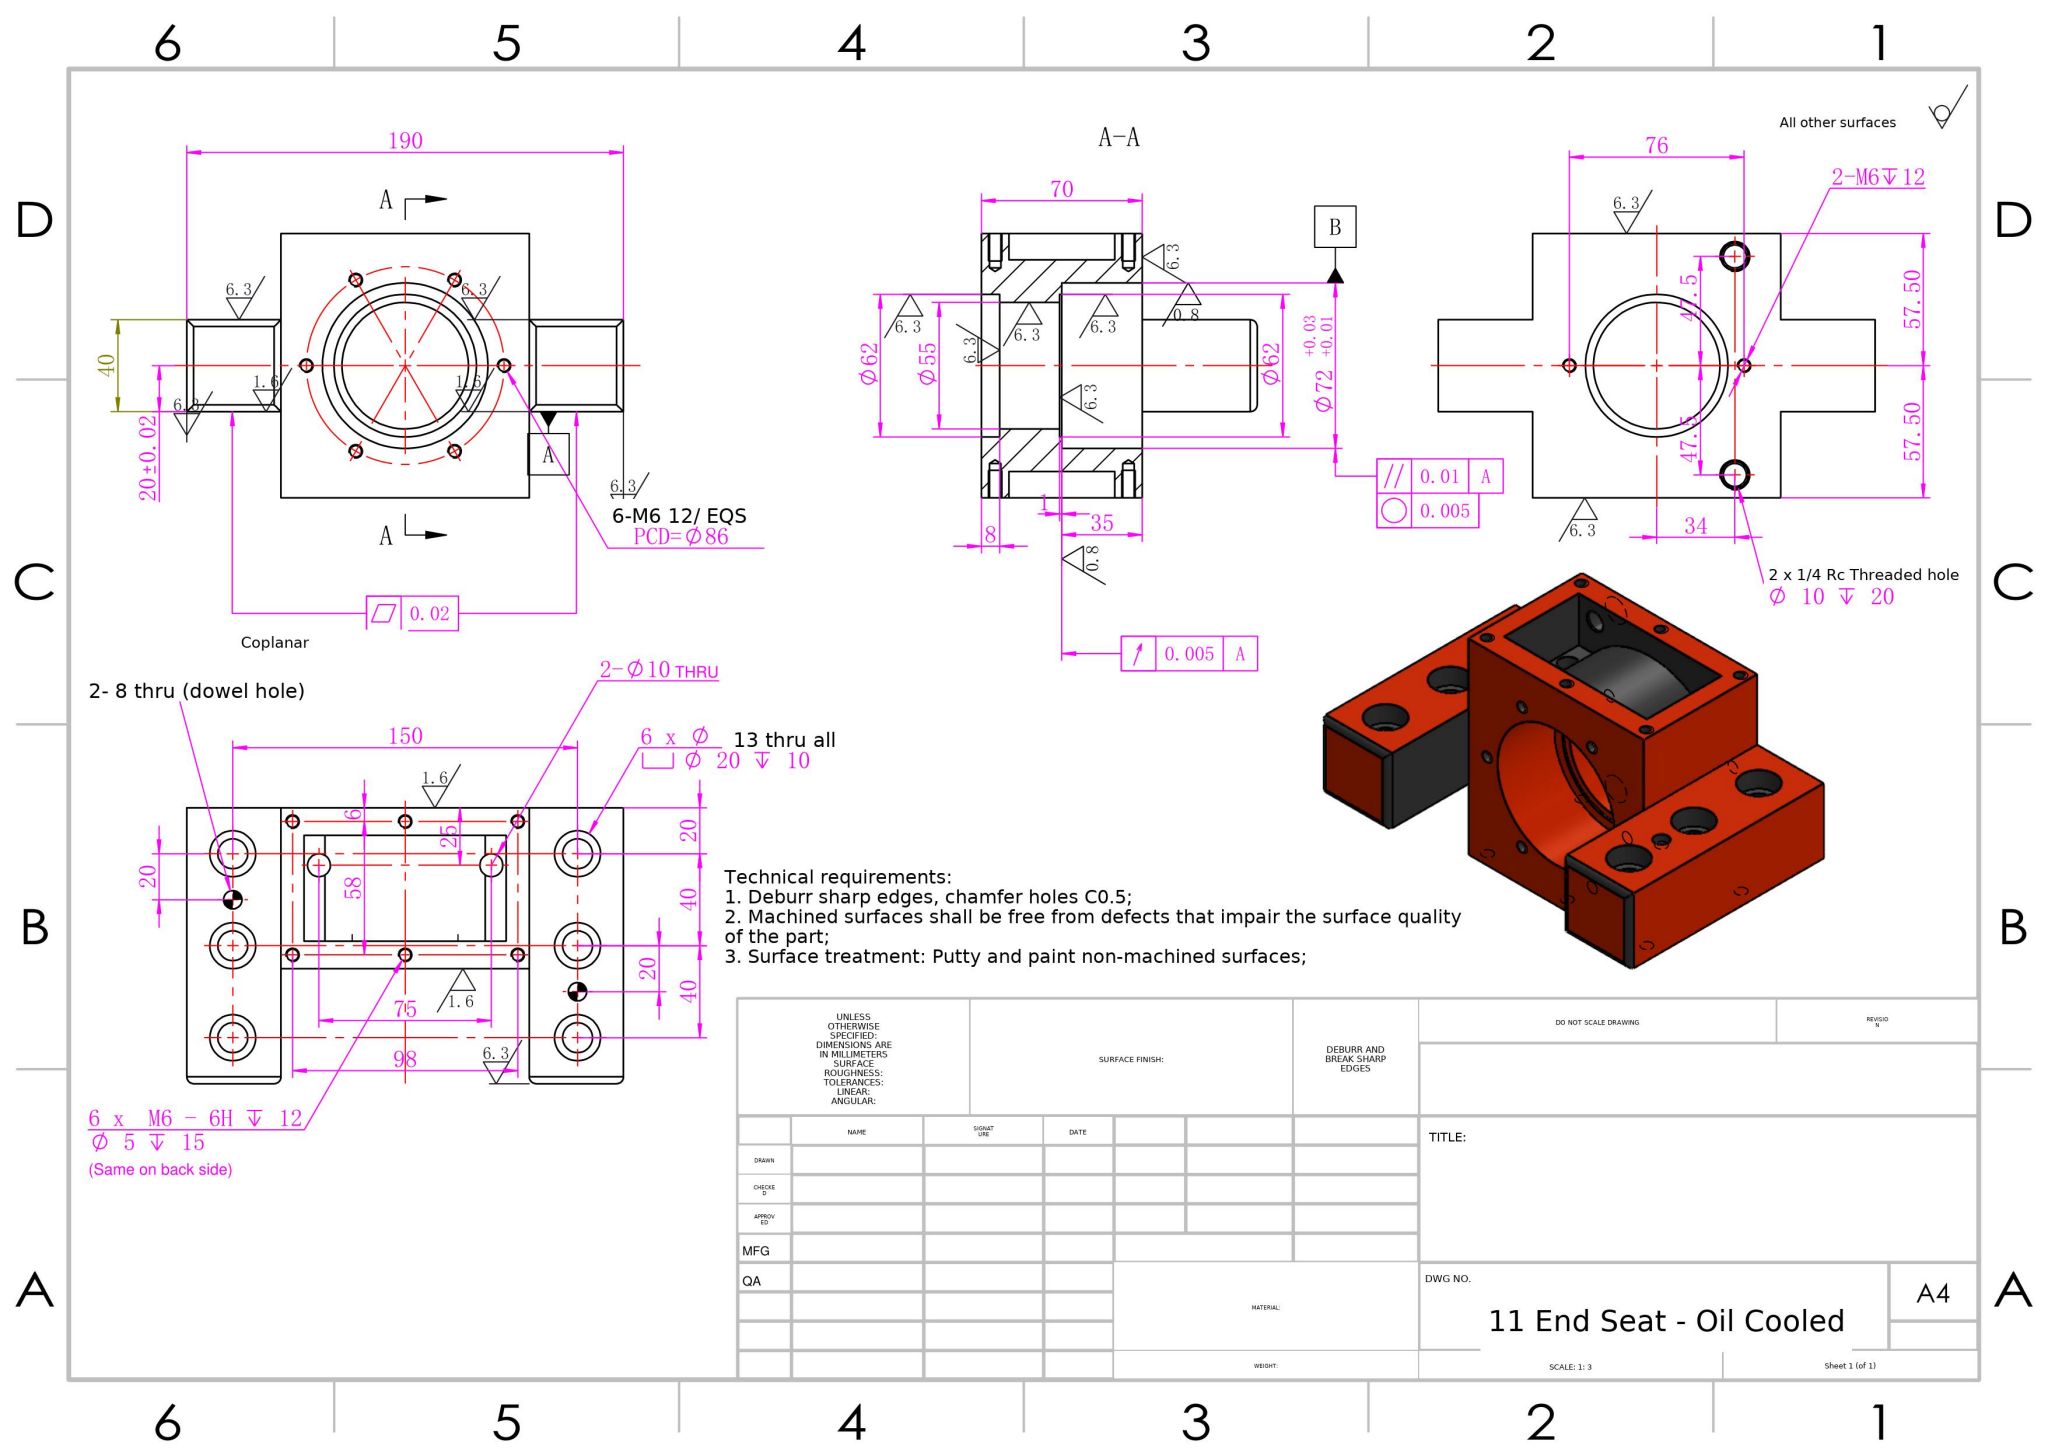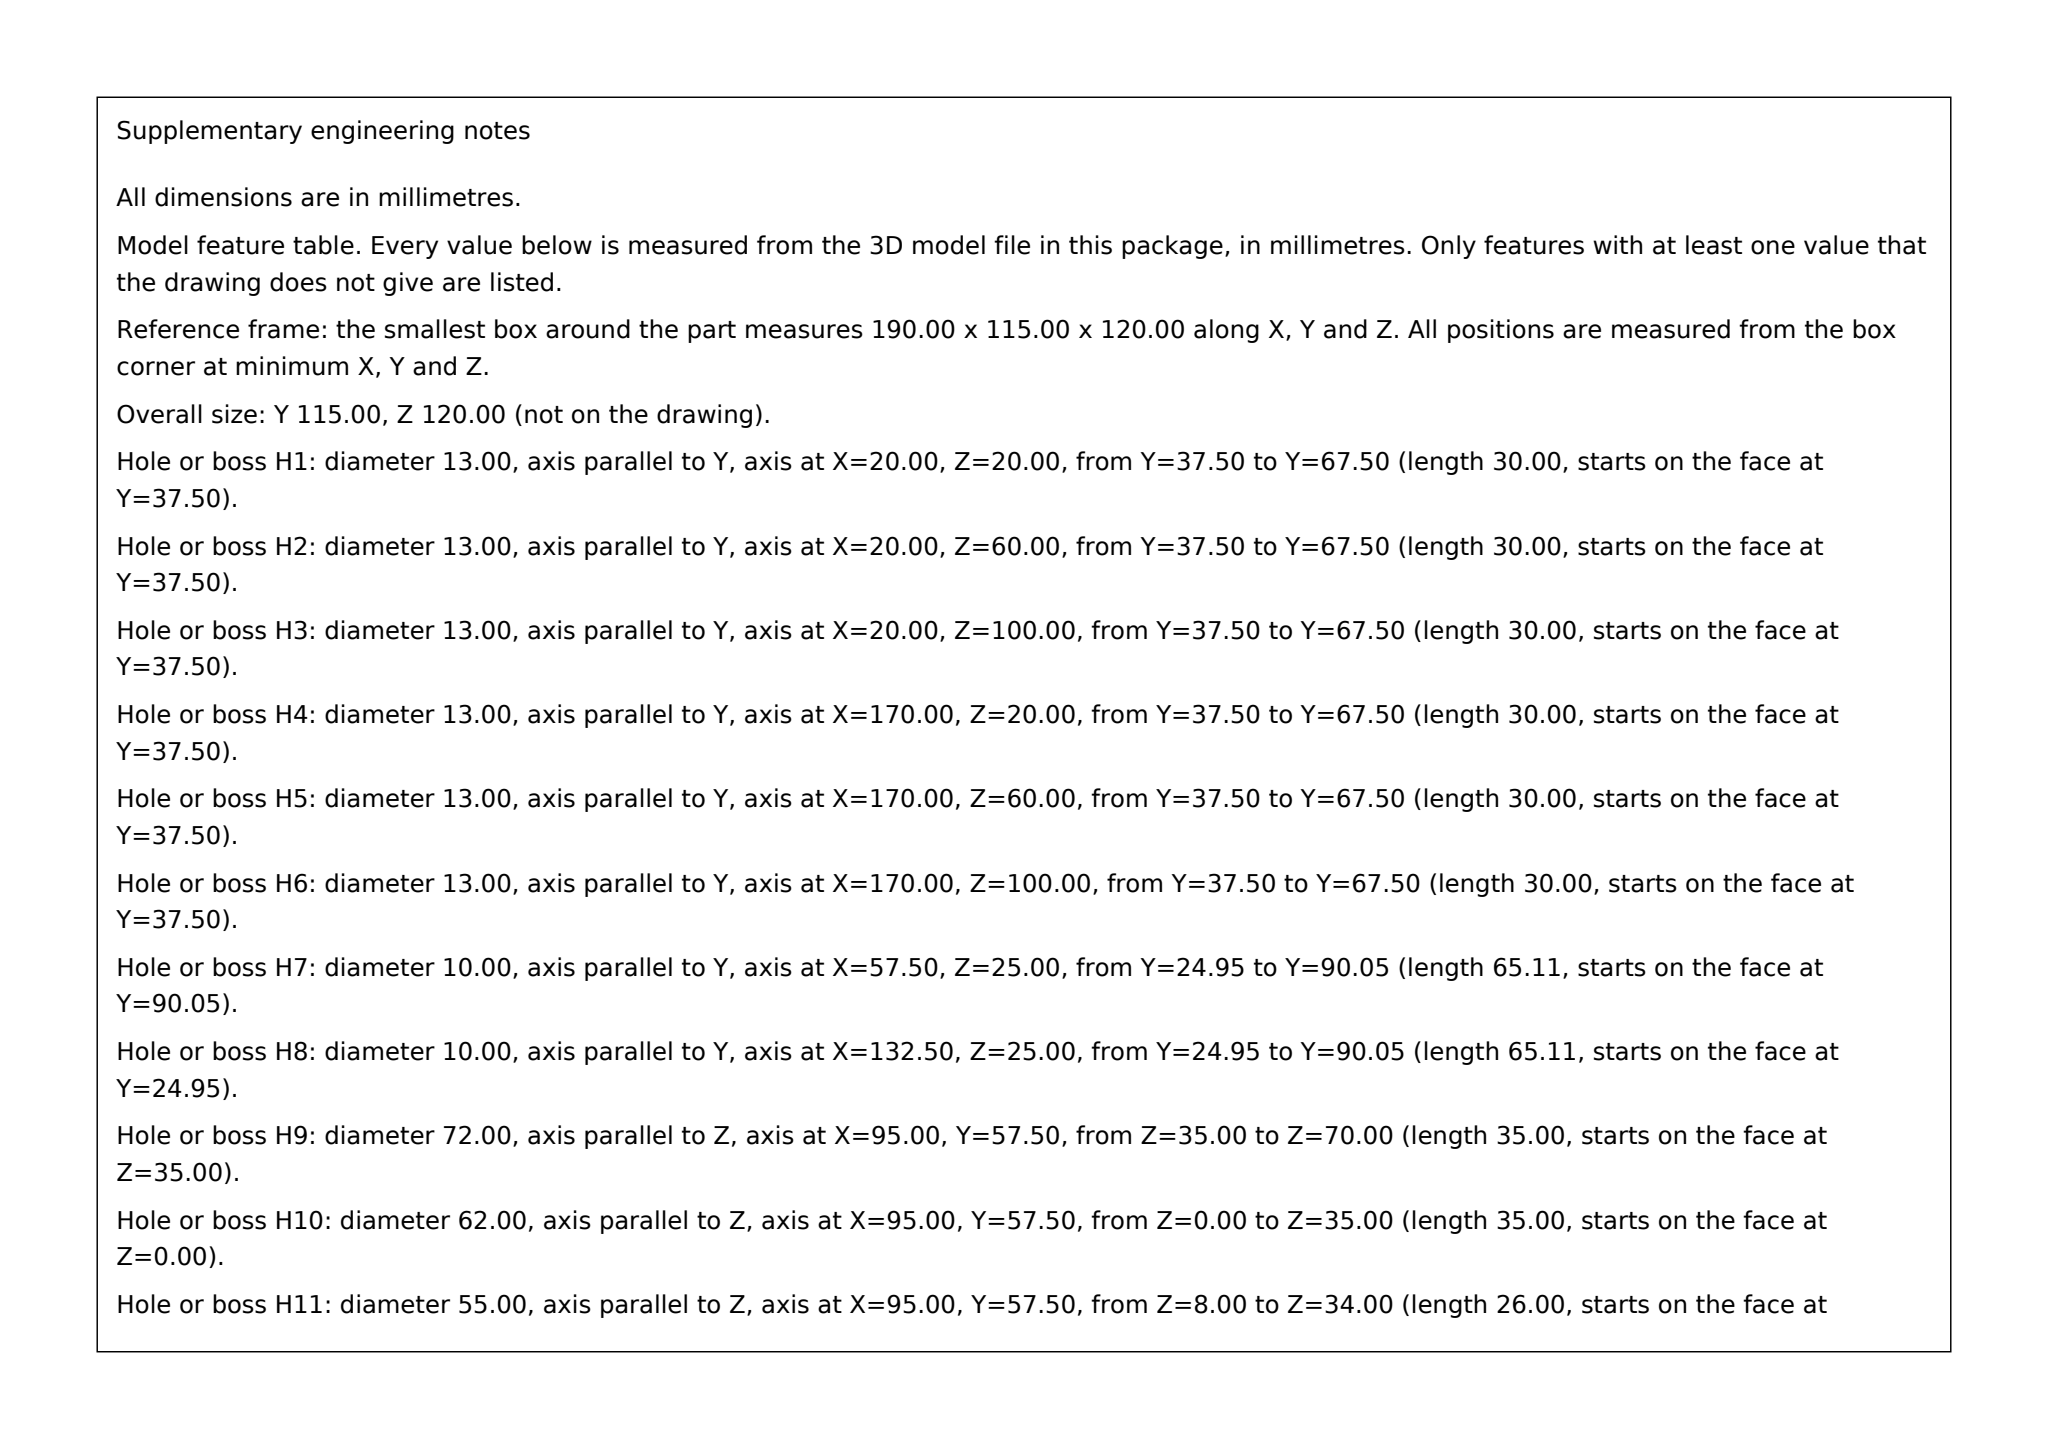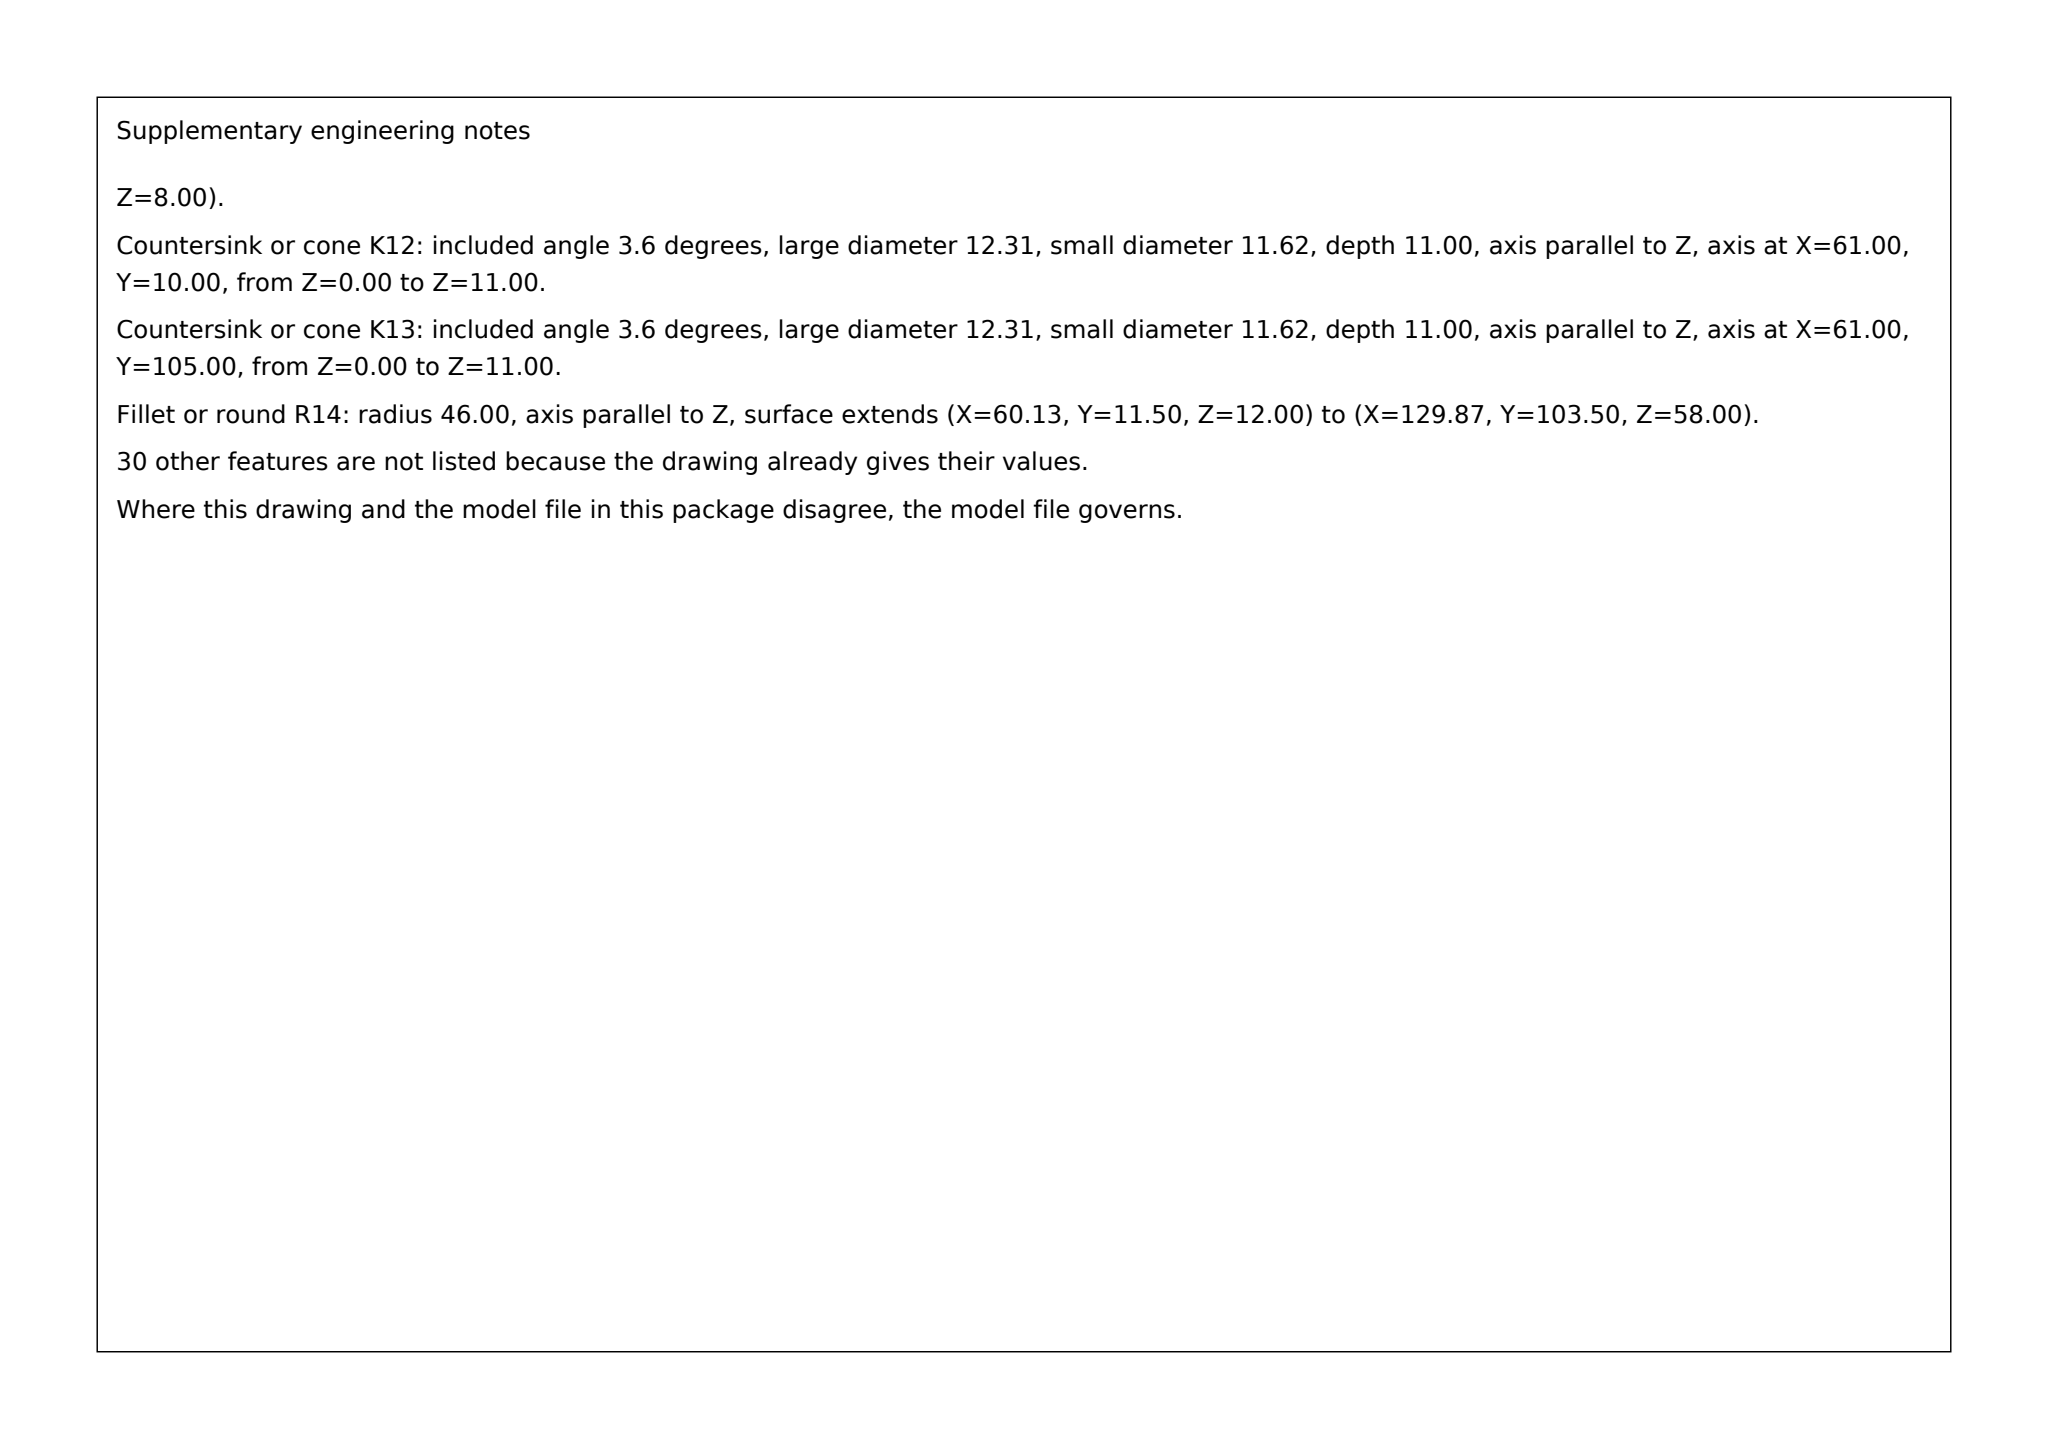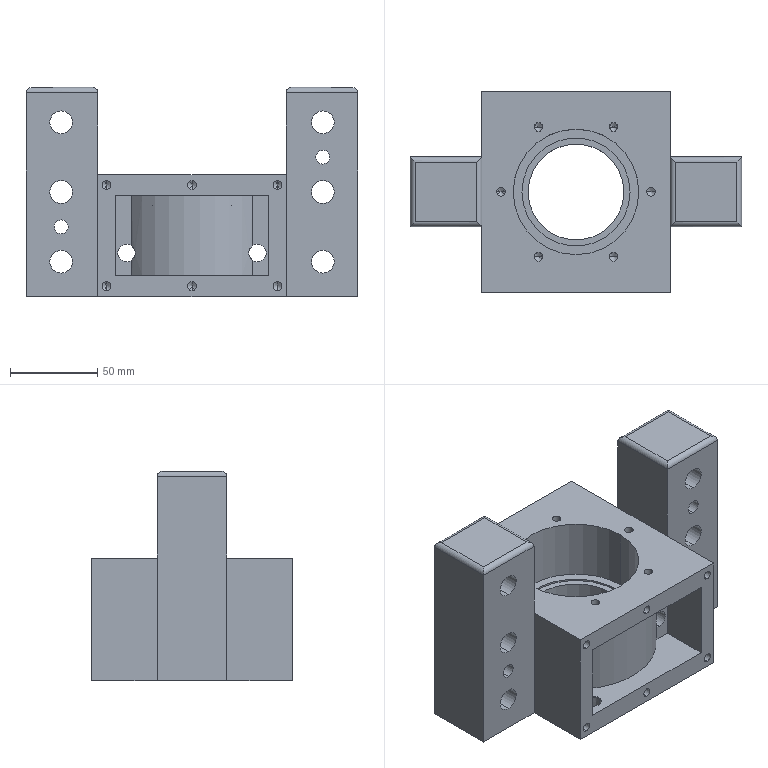Part | SolidWorks | mm | 1 solid | 179 faces | box 190 x 115 x 120 mm | volume 814112 mm3 | cylinder 94 | cone 44 | plane 41 | commonest cylinder face diameters 5 x40 20 x12 13 x12 10 x8 6 x8 8 x4 62 x4 72 x2
build123d program:
from build123d import *

# Parameters (mm, degrees)
SKETCH1_R                                            = 27.5
BOSS_EXTRUDE1_DEPTH                                  = 120
SKETCH3_W                                            = 108
SKETCH3_H                                            = 150
CUT_EXTRUDE1_DEPTH                                   = 50
SKETCH4_R                                            = 36
CUT_EXTRUDE2_DEPTH                                   = 35
SKETCH18_R                                           = 31
CUT_EXTRUDE7_DEPTH                                   = 8
CUT_EXTRUDE8_START                                   = -1
SKETCH19_R                                           = 31
CUT_EXTRUDE8_DEPTH                                   = 1
CYLINDRICAL_COUNTERSUNK_HOLE_FOR_M12_HEX_D           = 13
CYLINDRICAL_COUNTERSUNK_HOLE_FOR_M12_HEX_CBORE_D     = 20
CYLINDRICAL_COUNTERSUNK_HOLE_FOR_M12_HEX_CBORE_DEPTH = 10
CIRPATTERN1_COUNT                                    = 6
SIZE_MM_DOWEL_PIN_HOLE1_D                            = 8
M6_TAPPED_HOLE2_D                                    = 5
M6_TAPPED_HOLE2_DEPTH                                = 18
M6_TAPPED_HOLE2_TIP                                  = 1.502
BOSS_EXTRUDE2_REACH                                  = 187.607
SKETCH23_W                                           = 108
SKETCH23_H                                           = 70
BOSS_EXTRUDE3_REACH                                  = 193.442
SKETCH24_W                                           = 108
SKETCH24_H                                           = 70
SKETCH25_W                                           = 88
SKETCH25_H                                           = 46
CUT_EXTRUDE9_DEPTH                                   = 10
CUT_EXTRUDE10_DEPTH                                  = 46
SKETCH27_R                                           = 5
CUT_EXTRUDE11_DEPTH                                  = 192.442
M6_TAPPED_HOLE3_D                                    = 5
M6_TAPPED_HOLE3_DEPTH                                = 15
M6_TAPPED_HOLE3_TIP                                  = 1.502
M6_TAPPED_HOLE4_D                                    = 5
M6_TAPPED_HOLE4_DEPTH                                = 15
M6_TAPPED_HOLE4_TIP                                  = 1.502
F_1_4_RC_TAPPED_HOLE1_AT_2_COUNT                     = 2
F_1_4_RC_TAPPED_HOLE1_AT_2_PITCH                     = 95
FILLET1_R                                            = 3


with BuildPart() as part:
    # Sketch1 → Boss-Extrude1 (new body)
    with BuildSketch(Plane.XY):
        with BuildLine():
            Line((-95, 20), (-51.235, 20))
            ThreePointArc((-51.235, 20), (-41.806, 35.738), (-27.726, 47.5))
            Line((-27.726, 47.5), (27.726, 47.5))
            ThreePointArc((27.726, 47.5), (41.806, 35.738), (51.235, 20))
            Line((51.235, 20), (95, 20))
            Line((95, 20), (95, -20))
            Line((95, -20), (51.235, -20))
            ThreePointArc((51.235, -20), (41.806, -35.738), (27.726, -47.5))
            Line((27.726, -47.5), (-27.726, -47.5))
            ThreePointArc((-27.726, -47.5), (-41.806, -35.738), (-51.235, -20))
            Line((-51.235, -20), (-95, -20))
            Line((-95, -20), (-95, 20))
        make_face()
        Circle(SKETCH1_R, mode=Mode.SUBTRACT)
    extrude(amount=BOSS_EXTRUDE1_DEPTH)

    # Sketch3 → Cut-Extrude1 (cut)
    with BuildSketch(Plane.XY.offset(120)):
        Rectangle(SKETCH3_W, SKETCH3_H)
    extrude(amount=-CUT_EXTRUDE1_DEPTH, mode=Mode.SUBTRACT)

    # Sketch4 → Cut-Extrude2 (cut)
    with BuildSketch(Plane.XY.offset(70)):
        Circle(SKETCH4_R)
    extrude(amount=-CUT_EXTRUDE2_DEPTH, mode=Mode.SUBTRACT)

    # Sketch18 → Cut-Extrude7 (cut)
    with BuildSketch(Plane(origin=(0, 0, 0), x_dir=(-1, 0, 0), z_dir=(0, 0, -1))):
        Circle(SKETCH18_R)
    extrude(amount=-CUT_EXTRUDE7_DEPTH, mode=Mode.SUBTRACT)

    # Sketch19 → Cut-Extrude8 (cut)
    with BuildSketch(Plane.XY.offset(35).offset(CUT_EXTRUDE8_START)):
        with Locations(Location((0, 0, 0), (0, 0, 180))):
            Circle(SKETCH19_R)
    extrude(amount=CUT_EXTRUDE8_DEPTH, mode=Mode.SUBTRACT)

    # Cylindrical Countersunk Hole for M12 Hex (through all)
    with Locations(Plane(origin=(-75, 20, 100), x_dir=(1, 0, 0), z_dir=(0, 1, 0))):
        with Locations((0, 0), (0, 40), (0, 80), (150, 0), (150, 40), (150, 80)):
            CounterBoreHole(CYLINDRICAL_COUNTERSUNK_HOLE_FOR_M12_HEX_D / 2, CYLINDRICAL_COUNTERSUNK_HOLE_FOR_M12_HEX_CBORE_D / 2, CYLINDRICAL_COUNTERSUNK_HOLE_FOR_M12_HEX_CBORE_DEPTH)

    # Sketch9 → M6 Tapped Hole1 (revolve, cut)
    with BuildSketch(Plane(origin=(43, 0, 70), x_dir=(0, -1, 0), z_dir=(1, 0, 0))):
        Polygon((0, 0), (0, 19.502), (2.5, 18), (2.5, 0), align=None)
    m6_tapped_hole1 = revolve(axis=Axis((43, 0, 76.35), (0, 0, -1)), mode=Mode.SUBTRACT)

    # CirPattern1: M6 Tapped Hole1 ×6 about axis
    cirpattern1_axis = Axis((0, 0, 0), (0, 0, 1))
    for i in range(1, CIRPATTERN1_COUNT):
        add(m6_tapped_hole1.rotate(cirpattern1_axis, i * 360 / CIRPATTERN1_COUNT), mode=Mode.SUBTRACT)

    # Size mm Dowel Pin Hole1 (through all)
    with Locations(Plane(origin=(-75, 20, 40), x_dir=(1, 0, 0), z_dir=(0, 1, 0))):
        with Locations((0, 0), (150, -40)):
            Hole(SIZE_MM_DOWEL_PIN_HOLE1_D / 2)

    # M6 Tapped Hole2
    with Locations(Plane(origin=(38, 0, 0), x_dir=(-1, 0, 0), z_dir=(0, 0, -1))):
        with Locations((0, 0), (76, 0)):
            Hole(M6_TAPPED_HOLE2_D / 2, depth=M6_TAPPED_HOLE2_DEPTH)
            with Locations((0, 0, -(M6_TAPPED_HOLE2_DEPTH + M6_TAPPED_HOLE2_TIP / 2))):  # 118° drill point
                Cone(0, M6_TAPPED_HOLE2_D / 2, M6_TAPPED_HOLE2_TIP, mode=Mode.SUBTRACT)

    # Sketch23 → Boss-Extrude2 (add, up to next)
    with BuildSketch(Plane(origin=(0, 57.5, 0), x_dir=(1, 0, 0), z_dir=(0, 1, 0)), mode=Mode.PRIVATE) as boss_extrude2_sk1:
        with Locations((0, -35)):
            Rectangle(SKETCH23_W, SKETCH23_H)
    boss_extrude2_tool1 = extrude(boss_extrude2_sk1.sketch, amount=-BOSS_EXTRUDE2_REACH, mode=Mode.PRIVATE) - part.part
    add(boss_extrude2_tool1.solids().sort_by_distance((0, 57.5, 35))[0])

    # Sketch24 → Boss-Extrude3 (add, up to next)
    with BuildSketch(Plane(origin=(0, -57.5, 0), x_dir=(-1, 0, 0), z_dir=(0, -1, 0)), mode=Mode.PRIVATE) as boss_extrude3_sk1:
        with Locations((0, -35)):
            Rectangle(SKETCH24_W, SKETCH24_H)
    boss_extrude3_tool1 = extrude(boss_extrude3_sk1.sketch, amount=-BOSS_EXTRUDE3_REACH, mode=Mode.PRIVATE) - part.part
    add(boss_extrude3_tool1.solids().sort_by_distance((0, -57.5, 35))[0])

    # Sketch25 → Cut-Extrude9 (cut)
    with BuildSketch(Plane(origin=(0, 57.5, 0), x_dir=(1, 0, 0), z_dir=(0, 1, 0))):
        with Locations((0, -35)):
            Rectangle(SKETCH25_W, SKETCH25_H)
    extrude(amount=-CUT_EXTRUDE9_DEPTH, mode=Mode.SUBTRACT)

    # Sketch26 → Cut-Extrude10 (cut)
    with BuildSketch(Plane.XY.offset(12)):
        with BuildLine():
            Line((-44, 57.5), (-44, 30))
            Line((-44, 30), (-34.871, 30))
            ThreePointArc((-34.871, 30), (0, 46), (34.871, 30))
            Line((34.871, 30), (44, 30))
            Line((44, 30), (44, 57.5))
            Line((44, 57.5), (-44, 57.5))
        make_face()
        with BuildLine():
            Line((-44, -57.5), (44, -57.5))
            Line((44, -57.5), (44, -30))
            Line((44, -30), (34.871, -30))
            ThreePointArc((34.871, -30), (0, -46), (-34.871, -30))
            Line((-34.871, -30), (-44, -30))
            Line((-44, -30), (-44, -57.5))
        make_face()
    extrude(amount=CUT_EXTRUDE10_DEPTH, mode=Mode.SUBTRACT)

    # Sketch27 → Cut-Extrude11 (cut, through all)
    with BuildSketch(Plane(origin=(0, 57.5, 0), x_dir=(1, 0, 0), z_dir=(0, 1, 0))):
        with Locations(Location((-37.5, -25, 0), (0, 0, 58.28))):
            Circle(SKETCH27_R)
        with Locations(Location((37.5, -25, 0), (0, 0, 238.28))):
            Circle(SKETCH27_R)
    extrude(amount=-CUT_EXTRUDE11_DEPTH, mode=Mode.SUBTRACT)

    # M6 Tapped Hole3
    with Locations(Plane(origin=(0, 57.5, 0), x_dir=(1, 0, 0), z_dir=(0, 1, 0))):
        with Locations((-49, -6), (0, -6), (49, -6), (49, -64), (0, -64), (-49, -64)):
            Hole(M6_TAPPED_HOLE3_D / 2, depth=M6_TAPPED_HOLE3_DEPTH)
            with Locations((0, 0, -(M6_TAPPED_HOLE3_DEPTH + M6_TAPPED_HOLE3_TIP / 2))):  # 118° drill point
                Cone(0, M6_TAPPED_HOLE3_D / 2, M6_TAPPED_HOLE3_TIP, mode=Mode.SUBTRACT)

    # M6 Tapped Hole4
    with Locations(Plane(origin=(0, -57.5, 0), x_dir=(-1, 0, 0), z_dir=(0, -1, 0))):
        with Locations((-49, -6), (0, -6), (49, -6), (49, -64), (0, -64), (-49, -64)):
            Hole(M6_TAPPED_HOLE4_D / 2, depth=M6_TAPPED_HOLE4_DEPTH)
            with Locations((0, 0, -(M6_TAPPED_HOLE4_DEPTH + M6_TAPPED_HOLE4_TIP / 2))):  # 118° drill point
                Cone(0, M6_TAPPED_HOLE4_D / 2, M6_TAPPED_HOLE4_TIP, mode=Mode.SUBTRACT)

    # Sketch33 → 1_4 Rc Tapped Hole1 (revolve, cut)
    with BuildSketch(Plane(origin=(-34, 47.5, 0), x_dir=(0, 1, 0), z_dir=(1, 0, 0))):
        Polygon((0, 0), (0, 23.004), (5, 20), (5, 11), (5.811, 11), (6.154, 0), align=None)
    f_1_4_rc_tapped_hole1 = revolve(axis=Axis((-34, 47.5, -6.35), (0, 0, 1)), mode=Mode.SUBTRACT)

    # 1_4 Rc Tapped Hole1 at 2: 1_4 Rc Tapped Hole1 ×2
    with Locations(*[(0, -i * F_1_4_RC_TAPPED_HOLE1_AT_2_PITCH, 0) for i in range(1, F_1_4_RC_TAPPED_HOLE1_AT_2_COUNT)]):
        add(f_1_4_rc_tapped_hole1, mode=Mode.SUBTRACT)

    # Fillet1
    fillet1_edges = [part.edges().sort_by_distance(p)[0] for p in [
        (95, 0, 120),
        (74.5, 20, 120),
        (-74.5, 20, 120),
        (74.5, -20, 120),
        (-95, 0, 120),
        (-54, 0, 120),
        (54, 0, 120),
        (-74.5, -20, 120),
    ]]
    fillet(fillet1_edges, radius=FILLET1_R)


solid = part.part